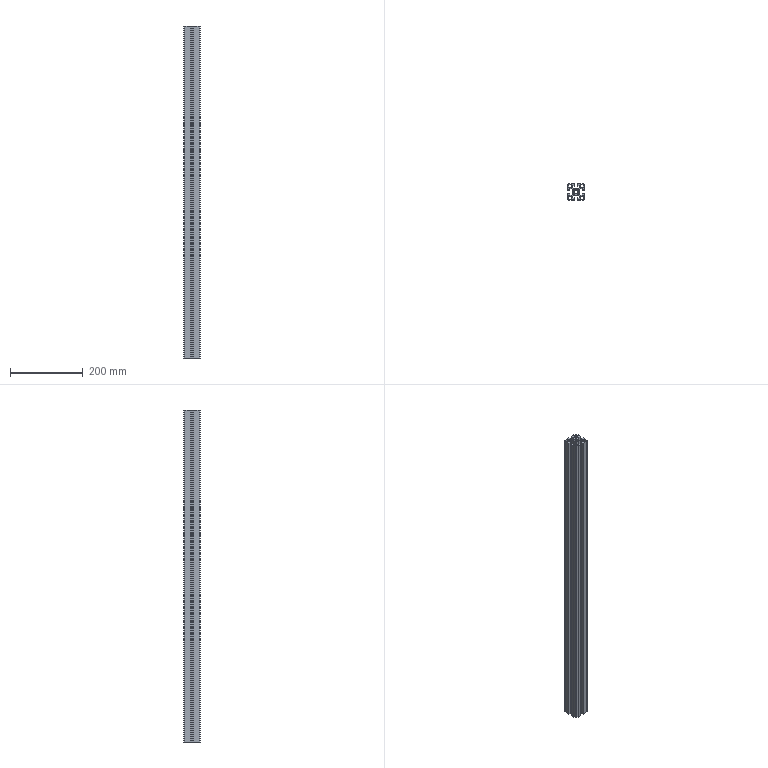Component | SolidWorks | 40-40AluminumProfileFrame-1_CAF8-4545-100GG-4 | 1 solid | 131 faces | volume 715237 mm3 | plane 82 | cylinder 49 | commonest cylinder face diameters 2 x18 3 x12 1 x10 12.5 x5 6 x4